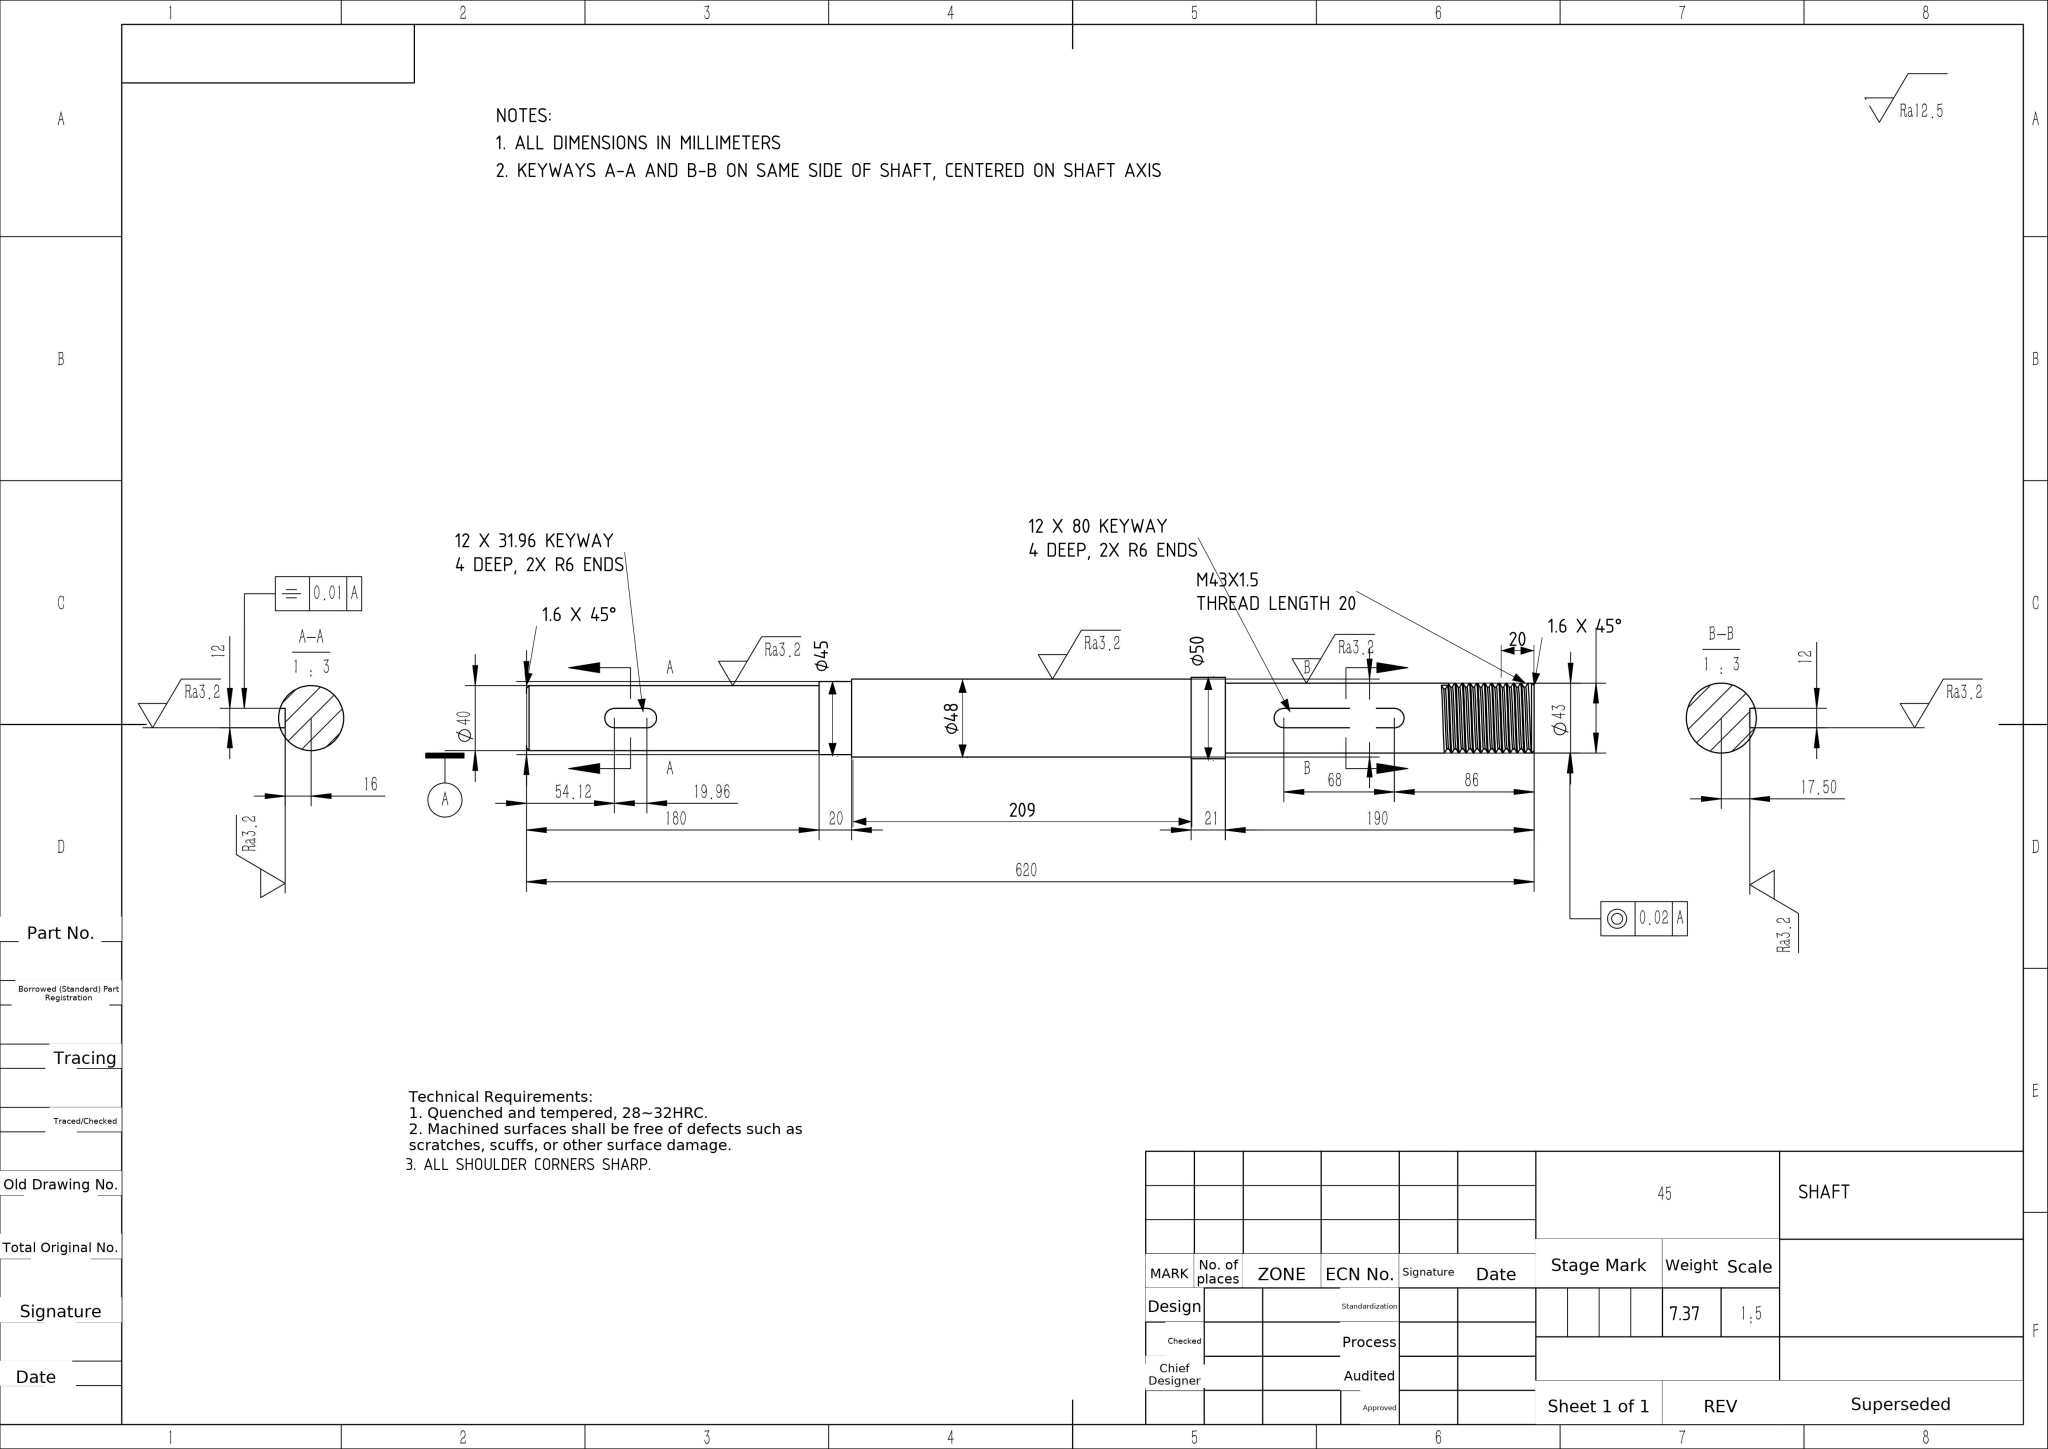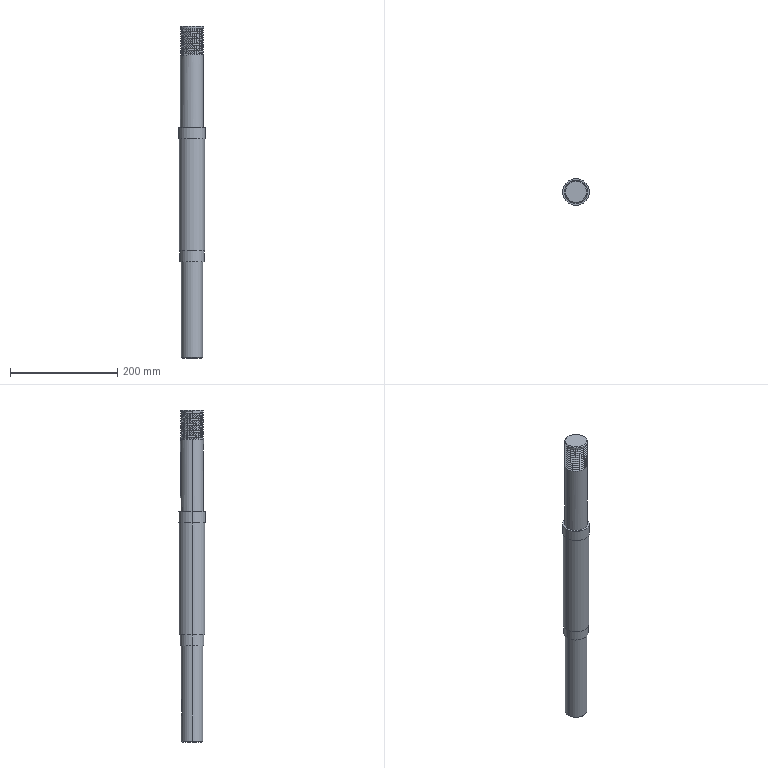Part | NX | mm | 1 solid | 59 faces | box 50 x 50 x 620 mm | volume 939021 mm3 | cylinder 38 | plane 14 | cone 4 | spline 3 | commonest cylinder face diameters 43 x24 12 x6 50 x2 48 x2 45 x2 40 x2